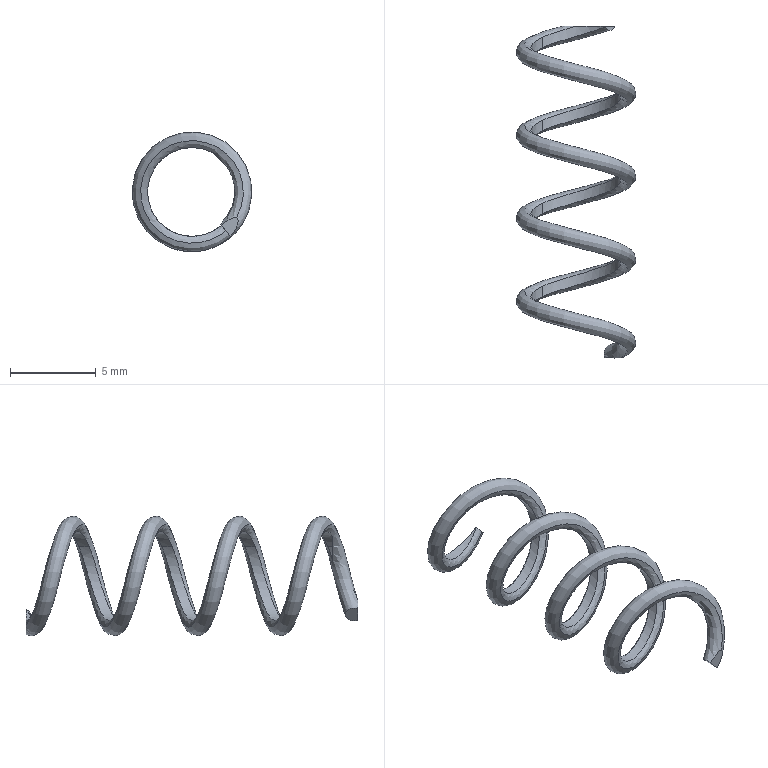Component | SolidWorks | VUM5-30-4 | 1 solid | 16 faces | volume 56 mm3 | cylinder 9 | plane 5 | spline 2 | commonest cylinder face diameters 5.2 x9